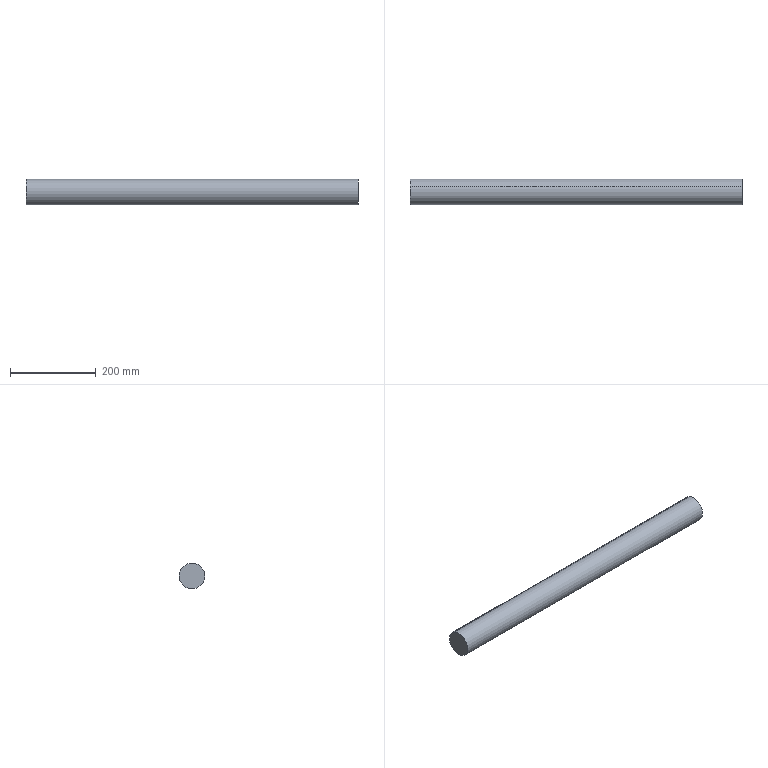Component | SolidWorks | SpindleBody-1 | 1 solid | 4 faces | box 772.78 x 60 x 60 mm | volume 2184983 mm3 | cylinder 2 | plane 2 | commonest cylinder face diameters 60 x2
build123d program:
from build123d import *

# Parameters (mm, degrees)
SKETCH1_W                         = 30
SKETCH1_H                         = 824.927
SKETCH2_R                         = 31
REPAIR_SEATINDRIVESHAFTBORE_DEPTH = 26.694


with BuildPart() as part:
    # Sketch1 → Revolve1 (revolve)
    with BuildSketch(Plane.XZ, mode=Mode.PRIVATE) as revolve1_sk:
        with Locations((-65.53, -159.684)):
            Rectangle(SKETCH1_W, SKETCH1_H)
    revolve(revolve1_sk.sketch.rotate(Axis((-80.53, 0, 252.78), (0, 0, -1)), 180), axis=Axis((-80.53, 0, 252.78), (0, 0, -1)))

    # Sketch2 → Repair_SeatInDriveShaftBore (cut, symmetric)
    with BuildSketch(Plane.XY.offset(-546.694)):
        with Locations((-80.53, 0)):
            Circle(SKETCH2_R)
    extrude(amount=REPAIR_SEATINDRIVESHAFTBORE_DEPTH, both=True, mode=Mode.SUBTRACT)


solid = part.part

# Placed as in the assembly
solid = solid.moved(Location((-232.112, 1335.766, 934.067), (0, 90, 0)))
STEP:
#1=COLOUR_RGB('',0.7922,0.8196,0.9333);
#2=FILL_AREA_STYLE_COLOUR('',#1);
#3=FILL_AREA_STYLE('',(#2));
#4=SURFACE_STYLE_FILL_AREA(#3);
#5=SURFACE_SIDE_STYLE('',(#4));
#6=SURFACE_STYLE_USAGE(.BOTH.,#5);
#7=PRESENTATION_STYLE_ASSIGNMENT((#6));
#8=CARTESIAN_POINT('',(0.8137,52.081,38.879));
#9=VERTEX_POINT('',#8);
#10=CARTESIAN_POINT('',(0.8137,53.098,41.011));
#11=VERTEX_POINT('',#10);
#12=CARTESIAN_POINT('',(0.8137,52.589,39.945));
#13=DIRECTION('',(-1.,0.,0.));
#14=DIRECTION('',(0.,-0.4306,-0.9025));
#15=AXIS2_PLACEMENT_3D('',#12,#13,#14);
#16=CIRCLE('',#15,1.181);
#17=EDGE_CURVE('',#9,#11,#16,.T.);
#18=ORIENTED_EDGE('',*,*,#17,.T.);
#19=CARTESIAN_POINT('',(-29.611,53.098,41.011));
#20=VERTEX_POINT('',#19);
#21=CARTESIAN_POINT('',(0.8137,53.098,41.011));
#22=DIRECTION('',(-1.,0.,0.));
#23=VECTOR('',#22,39.37);
#24=LINE('',#21,#23);
#25=EDGE_CURVE('',#11,#20,#24,.T.);
#26=ORIENTED_EDGE('',*,*,#25,.T.);
#27=CARTESIAN_POINT('',(-29.611,52.081,38.879));
#28=VERTEX_POINT('',#27);
#29=CARTESIAN_POINT('',(-29.611,52.589,39.945));
#30=DIRECTION('',(-1.,0.,0.));
#31=DIRECTION('',(0.,0.4306,0.9025));
#32=AXIS2_PLACEMENT_3D('',#29,#30,#31);
#33=CIRCLE('',#32,1.181);
#34=EDGE_CURVE('',#28,#20,#33,.T.);
#35=ORIENTED_EDGE('',*,*,#34,.F.);
#36=CARTESIAN_POINT('',(0.8137,52.081,38.879));
#37=DIRECTION('',(-1.,0.,0.));
#38=VECTOR('',#37,39.37);
#39=LINE('',#36,#38);
#40=EDGE_CURVE('',#9,#28,#39,.T.);
#41=ORIENTED_EDGE('',*,*,#40,.F.);
#42=EDGE_LOOP('',(#18,#26,#35,#41));
#43=FACE_OUTER_BOUND('',#42,.T.);
#44=CARTESIAN_POINT('',(0.8137,52.589,39.945));
#45=DIRECTION('',(-1.,0.,0.));
#46=DIRECTION('',(0.,-0.4306,-0.9025));
#47=AXIS2_PLACEMENT_3D('',#44,#45,#46);
#48=CYLINDRICAL_SURFACE('',#47,1.181);
#49=ADVANCED_FACE('',(#43),#48,.T.);
#50=ORIENTED_EDGE('',*,*,#25,.F.);
#51=CARTESIAN_POINT('',(0.8137,52.589,39.945));
#52=DIRECTION('',(-1.,0.,0.));
#53=DIRECTION('',(0.,-0.4306,-0.9025));
#54=AXIS2_PLACEMENT_3D('',#51,#52,#53);
#55=CIRCLE('',#54,1.181);
#56=EDGE_CURVE('',#11,#9,#55,.T.);
#57=ORIENTED_EDGE('',*,*,#56,.T.);
#58=ORIENTED_EDGE('',*,*,#40,.T.);
#59=CARTESIAN_POINT('',(-29.611,52.589,39.945));
#60=DIRECTION('',(-1.,0.,0.));
#61=DIRECTION('',(0.,0.4306,0.9025));
#62=AXIS2_PLACEMENT_3D('',#59,#60,#61);
#63=CIRCLE('',#62,1.181);
#64=EDGE_CURVE('',#20,#28,#63,.T.);
#65=ORIENTED_EDGE('',*,*,#64,.F.);
#66=EDGE_LOOP('',(#50,#57,#58,#65));
#67=FACE_OUTER_BOUND('',#66,.T.);
#68=CARTESIAN_POINT('',(0.8137,52.589,39.945));
#69=DIRECTION('',(-1.,0.,0.));
#70=DIRECTION('',(0.,-0.4306,-0.9025));
#71=AXIS2_PLACEMENT_3D('',#68,#69,#70);
#72=CYLINDRICAL_SURFACE('',#71,1.181);
#73=ADVANCED_FACE('',(#67),#72,.T.);
#74=ORIENTED_EDGE('',*,*,#17,.F.);
#75=ORIENTED_EDGE('',*,*,#56,.F.);
#76=EDGE_LOOP('',(#74,#75));
#77=FACE_OUTER_BOUND('',#76,.T.);
#78=CARTESIAN_POINT('',(0.8137,53.098,41.011));
#79=DIRECTION('',(1.,0.,0.));
#80=DIRECTION('',(0.,0.4306,0.9025));
#81=AXIS2_PLACEMENT_3D('',#78,#79,#80);
#82=PLANE('',#81);
#83=ADVANCED_FACE('',(#77),#82,.T.);
#84=ORIENTED_EDGE('',*,*,#34,.T.);
#85=ORIENTED_EDGE('',*,*,#64,.T.);
#86=EDGE_LOOP('',(#84,#85));
#87=FACE_OUTER_BOUND('',#86,.T.);
#88=CARTESIAN_POINT('',(-29.611,52.589,39.945));
#89=DIRECTION('',(1.,0.,0.));
#90=DIRECTION('',(0.,0.4306,0.9025));
#91=AXIS2_PLACEMENT_3D('',#88,#89,#90);
#92=PLANE('',#91);
#93=ADVANCED_FACE('',(#87),#92,.F.);
#94=CLOSED_SHELL('',(#49,#73,#83,#93));
#95=MANIFOLD_SOLID_BREP('',#94);
#96=STYLED_ITEM('',(#7),#95);
#97=(LENGTH_UNIT()NAMED_UNIT(*)SI_UNIT($,.METRE.));
#98=LENGTH_MEASURE_WITH_UNIT(LENGTH_MEASURE(0.0254),#97);
#99=DIMENSIONAL_EXPONENTS(1.,0.,0.,0.,0.,0.,0.);
#100=(CONVERSION_BASED_UNIT('',#98)LENGTH_UNIT()NAMED_UNIT(#99));
#101=UNCERTAINTY_MEASURE_WITH_UNIT(LENGTH_MEASURE(0.00001),#100,'','');
#102=(NAMED_UNIT(*)PLANE_ANGLE_UNIT()SI_UNIT($,.RADIAN.));
#103=(NAMED_UNIT(*)SI_UNIT($,.STERADIAN.)SOLID_ANGLE_UNIT());
#104=(GEOMETRIC_REPRESENTATION_CONTEXT(3)GLOBAL_UNCERTAINTY_ASSIGNED_CONTEXT((#101))GLOBAL_UNIT_ASSIGNED_CONTEXT((#100,#102,#103))REPRESENTATION_CONTEXT('',''));
#105=MECHANICAL_DESIGN_GEOMETRIC_PRESENTATION_REPRESENTATION('',(#96),#104);
#106=CARTESIAN_POINT('',(0.,0.,0.));
#107=DIRECTION('',(0.,0.,1.));
#108=DIRECTION('',(1.,0.,0.));
#109=AXIS2_PLACEMENT_3D('',#106,#107,#108);
#110=(LENGTH_UNIT()NAMED_UNIT(*)SI_UNIT($,.METRE.));
#111=LENGTH_MEASURE_WITH_UNIT(LENGTH_MEASURE(0.0254),#110);
#112=DIMENSIONAL_EXPONENTS(1.,0.,0.,0.,0.,0.,0.);
#113=(CONVERSION_BASED_UNIT('',#111)LENGTH_UNIT()NAMED_UNIT(#112));
#114=UNCERTAINTY_MEASURE_WITH_UNIT(LENGTH_MEASURE(0.00001),#113,'','');
#115=(NAMED_UNIT(*)PLANE_ANGLE_UNIT()SI_UNIT($,.RADIAN.));
#116=(NAMED_UNIT(*)SI_UNIT($,.STERADIAN.)SOLID_ANGLE_UNIT());
#117=(GEOMETRIC_REPRESENTATION_CONTEXT(3)GLOBAL_UNCERTAINTY_ASSIGNED_CONTEXT((#114))GLOBAL_UNIT_ASSIGNED_CONTEXT((#113,#115,#116))REPRESENTATION_CONTEXT('',''));
#118=ADVANCED_BREP_SHAPE_REPRESENTATION('',(#95,#109),#117);
#119=PRESENTATION_LAYER_ASSIGNMENT('','',(#96));